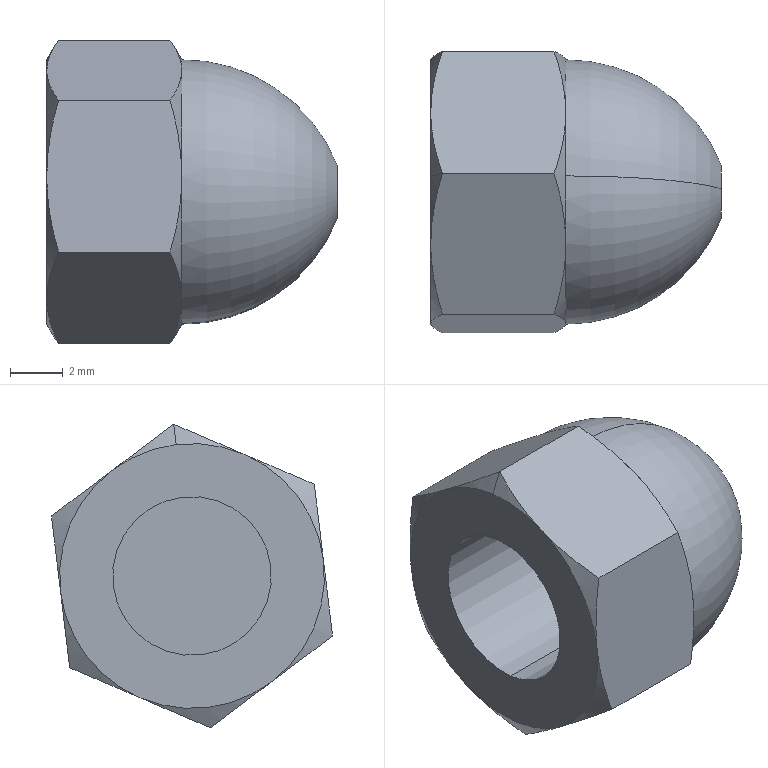Component | SolidWorks | DNR-71M20100BBEF2xx-A_990608MSS-1 | 1 solid | 26 faces | box 10.97 x 10.62 x 11.46 mm | volume 572 mm3 | cone 13 | plane 9 | torus 2 | cylinder 2 | commonest cylinder face diameters 6 x2
STEP:
#1=COLOUR_RGB('',0.7922,0.8196,0.9333);
#2=FILL_AREA_STYLE_COLOUR('',#1);
#3=FILL_AREA_STYLE('',(#2));
#4=SURFACE_STYLE_FILL_AREA(#3);
#5=SURFACE_SIDE_STYLE('',(#4));
#6=SURFACE_STYLE_USAGE(.BOTH.,#5);
#7=PRESENTATION_STYLE_ASSIGNMENT((#6));
#8=CARTESIAN_POINT('',(11.05,-7.185,8.11));
#9=VERTEX_POINT('',#8);
#10=CARTESIAN_POINT('',(11.05,-7.091,8.072));
#11=VERTEX_POINT('',#10);
#12=CARTESIAN_POINT('',(11.05,-7.067,8.267));
#13=DIRECTION('',(1.,-0.,-0.));
#14=DIRECTION('',(-0.,-0.9928,0.1196));
#15=AXIS2_PLACEMENT_3D('',#12,#13,#14);
#16=CIRCLE('',#15,0.1969);
#17=EDGE_CURVE('',#9,#11,#16,.T.);
#18=ORIENTED_EDGE('',*,*,#17,.T.);
#19=CARTESIAN_POINT('',(11.281,-7.072,8.227));
#20=VERTEX_POINT('',#19);
#21=CARTESIAN_POINT('',(11.05,-7.061,8.319));
#22=DIRECTION('',(-0.,-0.9928,0.1196));
#23=DIRECTION('',(0.,-0.1196,-0.9928));
#24=AXIS2_PLACEMENT_3D('',#21,#22,#23);
#25=CIRCLE('',#24,0.2487);
#26=EDGE_CURVE('',#11,#20,#25,.T.);
#27=ORIENTED_EDGE('',*,*,#26,.T.);
#28=CARTESIAN_POINT('',(11.281,-7.062,8.307));
#29=VERTEX_POINT('',#28);
#30=CARTESIAN_POINT('',(11.281,-7.067,8.267));
#31=DIRECTION('',(-1.,0.,0.));
#32=DIRECTION('',(0.,0.1196,0.9928));
#33=AXIS2_PLACEMENT_3D('',#30,#31,#32);
#34=CIRCLE('',#33,0.04003);
#35=EDGE_CURVE('',#20,#29,#34,.T.);
#36=ORIENTED_EDGE('',*,*,#35,.T.);
#37=CARTESIAN_POINT('',(11.05,-7.044,8.463));
#38=VERTEX_POINT('',#37);
#39=CARTESIAN_POINT('',(11.05,-7.073,8.216));
#40=DIRECTION('',(0.,0.9928,-0.1196));
#41=DIRECTION('',(0.,0.1196,0.9928));
#42=AXIS2_PLACEMENT_3D('',#39,#40,#41);
#43=CIRCLE('',#42,0.2487);
#44=EDGE_CURVE('',#38,#29,#43,.T.);
#45=ORIENTED_EDGE('',*,*,#44,.F.);
#46=CARTESIAN_POINT('',(11.05,-7.144,8.448));
#47=VERTEX_POINT('',#46);
#48=CARTESIAN_POINT('',(11.05,-7.067,8.267));
#49=DIRECTION('',(1.,0.,0.));
#50=DIRECTION('',(0.,-0.9928,0.1196));
#51=AXIS2_PLACEMENT_3D('',#48,#49,#50);
#52=CIRCLE('',#51,0.1969);
#53=EDGE_CURVE('',#38,#47,#52,.T.);
#54=ORIENTED_EDGE('',*,*,#53,.T.);
#55=CARTESIAN_POINT('',(11.05,-7.263,8.291));
#56=VERTEX_POINT('',#55);
#57=CARTESIAN_POINT('',(11.05,-7.067,8.267));
#58=DIRECTION('',(1.,0.,0.));
#59=DIRECTION('',(0.,-0.9928,0.1196));
#60=AXIS2_PLACEMENT_3D('',#57,#58,#59);
#61=CIRCLE('',#60,0.1969);
#62=EDGE_CURVE('',#47,#56,#61,.T.);
#63=ORIENTED_EDGE('',*,*,#62,.T.);
#64=CARTESIAN_POINT('',(11.05,-7.067,8.267));
#65=DIRECTION('',(1.,-0.,-0.));
#66=DIRECTION('',(-0.,-0.9928,0.1196));
#67=AXIS2_PLACEMENT_3D('',#64,#65,#66);
#68=CIRCLE('',#67,0.1969);
#69=EDGE_CURVE('',#56,#9,#68,.T.);
#70=ORIENTED_EDGE('',*,*,#69,.T.);
#71=EDGE_LOOP('',(#18,#27,#36,#45,#54,#63,#70));
#72=FACE_OUTER_BOUND('',#71,.T.);
#73=CARTESIAN_POINT('',(11.05,-7.067,8.267));
#74=DIRECTION('',(1.,-0.,-0.));
#75=DIRECTION('',(0.,0.1196,0.9928));
#76=AXIS2_PLACEMENT_3D('',#73,#74,#75);
#77=TOROIDAL_SURFACE('',#76,-0.05184,0.2487);
#78=ADVANCED_FACE('',(#72),#77,.T.);
#79=CARTESIAN_POINT('',(10.849,-6.949,8.425));
#80=VERTEX_POINT('',#79);
#81=CARTESIAN_POINT('',(10.849,-7.044,8.463));
#82=VERTEX_POINT('',#81);
#83=CARTESIAN_POINT('',(10.849,-7.067,8.267));
#84=DIRECTION('',(1.,-0.,-0.));
#85=DIRECTION('',(0.,0.1196,0.9928));
#86=AXIS2_PLACEMENT_3D('',#83,#84,#85);
#87=CIRCLE('',#86,0.1969);
#88=EDGE_CURVE('',#80,#82,#87,.T.);
#89=ORIENTED_EDGE('',*,*,#88,.T.);
#90=CARTESIAN_POINT('',(10.867,-7.04,8.493));
#91=VERTEX_POINT('',#90);
#92=CARTESIAN_POINT('',(10.867,-7.04,8.493));
#93=DIRECTION('',(0.5,0.1036,0.8598));
#94=VECTOR('',#93,39.37);
#95=LINE('',#92,#94);
#96=EDGE_CURVE('',#82,#91,#95,.T.);
#97=ORIENTED_EDGE('',*,*,#96,.T.);
#98=CARTESIAN_POINT('',(10.849,-6.949,8.425));
#99=CARTESIAN_POINT('',(10.849,-6.98,8.448));
#100=CARTESIAN_POINT('',(10.856,-7.01,8.47));
#101=CARTESIAN_POINT('',(10.867,-7.04,8.493));
#102=B_SPLINE_CURVE_WITH_KNOTS('',3,(#98,#99,#100,#101),.UNSPECIFIED.,.F.,.F.,(4,4),(0.,0.002921),.UNSPECIFIED.);
#103=EDGE_CURVE('',#80,#91,#102,.T.);
#104=ORIENTED_EDGE('',*,*,#103,.F.);
#105=EDGE_LOOP('',(#89,#97,#104));
#106=FACE_OUTER_BOUND('',#105,.T.);
#107=CARTESIAN_POINT('',(10.867,-7.067,8.267));
#108=DIRECTION('',(1.,-0.,-0.));
#109=DIRECTION('',(0.,0.1196,0.9928));
#110=AXIS2_PLACEMENT_3D('',#107,#108,#109);
#111=CONICAL_SURFACE('',#110,0.2275,1.047);
#112=ADVANCED_FACE('',(#106),#111,.T.);
#113=CARTESIAN_POINT('',(10.849,-7.081,8.15));
#114=VERTEX_POINT('',#113);
#115=CARTESIAN_POINT('',(10.849,-7.053,8.384));
#116=VERTEX_POINT('',#115);
#117=CARTESIAN_POINT('',(10.849,-7.067,8.267));
#118=DIRECTION('',(1.,-0.,-0.));
#119=DIRECTION('',(0.,0.1196,0.9928));
#120=AXIS2_PLACEMENT_3D('',#117,#118,#119);
#121=CIRCLE('',#120,0.1181);
#122=EDGE_CURVE('',#114,#116,#121,.T.);
#123=ORIENTED_EDGE('',*,*,#122,.F.);
#124=CARTESIAN_POINT('',(11.086,-7.081,8.15));
#125=VERTEX_POINT('',#124);
#126=CARTESIAN_POINT('',(10.849,-7.081,8.15));
#127=DIRECTION('',(1.,-0.,-0.));
#128=VECTOR('',#127,39.37);
#129=LINE('',#126,#128);
#130=EDGE_CURVE('',#114,#125,#129,.T.);
#131=ORIENTED_EDGE('',*,*,#130,.T.);
#132=CARTESIAN_POINT('',(11.086,-7.053,8.384));
#133=VERTEX_POINT('',#132);
#134=CARTESIAN_POINT('',(11.086,-7.067,8.267));
#135=DIRECTION('',(-1.,0.,0.));
#136=DIRECTION('',(0.,0.1196,0.9928));
#137=AXIS2_PLACEMENT_3D('',#134,#135,#136);
#138=CIRCLE('',#137,0.1181);
#139=EDGE_CURVE('',#133,#125,#138,.T.);
#140=ORIENTED_EDGE('',*,*,#139,.F.);
#141=CARTESIAN_POINT('',(10.849,-7.053,8.384));
#142=DIRECTION('',(1.,-0.,-0.));
#143=VECTOR('',#142,39.37);
#144=LINE('',#141,#143);
#145=EDGE_CURVE('',#116,#133,#144,.T.);
#146=ORIENTED_EDGE('',*,*,#145,.F.);
#147=EDGE_LOOP('',(#123,#131,#140,#146));
#148=FACE_OUTER_BOUND('',#147,.T.);
#149=CARTESIAN_POINT('',(10.849,-7.067,8.267));
#150=DIRECTION('',(1.,-0.,-0.));
#151=DIRECTION('',(0.,0.1196,0.9928));
#152=AXIS2_PLACEMENT_3D('',#149,#150,#151);
#153=CYLINDRICAL_SURFACE('',#152,0.1181);
#154=ADVANCED_FACE('',(#148),#153,.F.);
#155=ORIENTED_EDGE('',*,*,#26,.F.);
#156=CARTESIAN_POINT('',(11.05,-6.99,8.086));
#157=VERTEX_POINT('',#156);
#158=CARTESIAN_POINT('',(11.05,-7.067,8.267));
#159=DIRECTION('',(1.,-0.,-0.));
#160=DIRECTION('',(-0.,-0.9928,0.1196));
#161=AXIS2_PLACEMENT_3D('',#158,#159,#160);
#162=CIRCLE('',#161,0.1969);
#163=EDGE_CURVE('',#11,#157,#162,.T.);
#164=ORIENTED_EDGE('',*,*,#163,.T.);
#165=CARTESIAN_POINT('',(11.05,-6.872,8.244));
#166=VERTEX_POINT('',#165);
#167=CARTESIAN_POINT('',(11.05,-7.067,8.267));
#168=DIRECTION('',(1.,-0.,-0.));
#169=DIRECTION('',(-0.,-0.9928,0.1196));
#170=AXIS2_PLACEMENT_3D('',#167,#168,#169);
#171=CIRCLE('',#170,0.1969);
#172=EDGE_CURVE('',#157,#166,#171,.T.);
#173=ORIENTED_EDGE('',*,*,#172,.T.);
#174=CARTESIAN_POINT('',(11.05,-6.949,8.425));
#175=VERTEX_POINT('',#174);
#176=CARTESIAN_POINT('',(11.05,-7.067,8.267));
#177=DIRECTION('',(1.,0.,0.));
#178=DIRECTION('',(0.,-0.9928,0.1196));
#179=AXIS2_PLACEMENT_3D('',#176,#177,#178);
#180=CIRCLE('',#179,0.1969);
#181=EDGE_CURVE('',#166,#175,#180,.T.);
#182=ORIENTED_EDGE('',*,*,#181,.T.);
#183=CARTESIAN_POINT('',(11.05,-7.067,8.267));
#184=DIRECTION('',(1.,0.,0.));
#185=DIRECTION('',(0.,-0.9928,0.1196));
#186=AXIS2_PLACEMENT_3D('',#183,#184,#185);
#187=CIRCLE('',#186,0.1969);
#188=EDGE_CURVE('',#175,#38,#187,.T.);
#189=ORIENTED_EDGE('',*,*,#188,.T.);
#190=ORIENTED_EDGE('',*,*,#44,.T.);
#191=CARTESIAN_POINT('',(11.281,-7.067,8.267));
#192=DIRECTION('',(-1.,0.,0.));
#193=DIRECTION('',(0.,0.1196,0.9928));
#194=AXIS2_PLACEMENT_3D('',#191,#192,#193);
#195=CIRCLE('',#194,0.04003);
#196=EDGE_CURVE('',#29,#20,#195,.T.);
#197=ORIENTED_EDGE('',*,*,#196,.T.);
#198=EDGE_LOOP('',(#155,#164,#173,#182,#189,#190,#197));
#199=FACE_OUTER_BOUND('',#198,.T.);
#200=CARTESIAN_POINT('',(11.05,-7.067,8.267));
#201=DIRECTION('',(1.,-0.,-0.));
#202=DIRECTION('',(0.,0.1196,0.9928));
#203=AXIS2_PLACEMENT_3D('',#200,#201,#202);
#204=TOROIDAL_SURFACE('',#203,-0.05184,0.2487);
#205=ADVANCED_FACE('',(#199),#204,.T.);
#206=ORIENTED_EDGE('',*,*,#196,.F.);
#207=ORIENTED_EDGE('',*,*,#35,.F.);
#208=EDGE_LOOP('',(#206,#207));
#209=FACE_OUTER_BOUND('',#208,.T.);
#210=CARTESIAN_POINT('',(11.281,-7.067,8.267));
#211=DIRECTION('',(1.,-0.,-0.));
#212=DIRECTION('',(0.,0.1196,0.9928));
#213=AXIS2_PLACEMENT_3D('',#210,#211,#212);
#214=PLANE('',#213);
#215=ADVANCED_FACE('',(#209),#214,.T.);
#216=CARTESIAN_POINT('',(11.033,-6.885,8.131));
#217=VERTEX_POINT('',#216);
#218=CARTESIAN_POINT('',(11.033,-6.885,8.131));
#219=CARTESIAN_POINT('',(11.043,-6.881,8.168));
#220=CARTESIAN_POINT('',(11.05,-6.876,8.205));
#221=CARTESIAN_POINT('',(11.05,-6.872,8.244));
#222=B_SPLINE_CURVE_WITH_KNOTS('',3,(#218,#219,#220,#221),.UNSPECIFIED.,.F.,.F.,(4,4),(0.,0.002921),.UNSPECIFIED.);
#223=EDGE_CURVE('',#217,#166,#222,.T.);
#224=ORIENTED_EDGE('',*,*,#223,.T.);
#225=ORIENTED_EDGE('',*,*,#172,.F.);
#226=CARTESIAN_POINT('',(11.05,-6.99,8.086));
#227=CARTESIAN_POINT('',(11.05,-6.954,8.101));
#228=CARTESIAN_POINT('',(11.043,-6.919,8.116));
#229=CARTESIAN_POINT('',(11.033,-6.885,8.131));
#230=B_SPLINE_CURVE_WITH_KNOTS('',3,(#226,#227,#228,#229),.UNSPECIFIED.,.F.,.F.,(4,4),(0.,0.002921),.UNSPECIFIED.);
#231=EDGE_CURVE('',#157,#217,#230,.T.);
#232=ORIENTED_EDGE('',*,*,#231,.T.);
#233=EDGE_LOOP('',(#224,#225,#232));
#234=FACE_OUTER_BOUND('',#233,.T.);
#235=CARTESIAN_POINT('',(11.032,-7.067,8.267));
#236=DIRECTION('',(-1.,0.,0.));
#237=DIRECTION('',(0.,0.9928,-0.1196));
#238=AXIS2_PLACEMENT_3D('',#235,#236,#237);
#239=CONICAL_SURFACE('',#238,0.2275,1.047);
#240=ADVANCED_FACE('',(#234),#239,.T.);
#241=CARTESIAN_POINT('',(11.033,-7.094,8.041));
#242=VERTEX_POINT('',#241);
#243=CARTESIAN_POINT('',(11.033,-7.094,8.041));
#244=CARTESIAN_POINT('',(11.043,-7.06,8.056));
#245=CARTESIAN_POINT('',(11.05,-7.025,8.071));
#246=CARTESIAN_POINT('',(11.05,-6.99,8.086));
#247=B_SPLINE_CURVE_WITH_KNOTS('',3,(#243,#244,#245,#246),.UNSPECIFIED.,.F.,.F.,(4,4),(0.,0.002921),.UNSPECIFIED.);
#248=EDGE_CURVE('',#242,#157,#247,.T.);
#249=ORIENTED_EDGE('',*,*,#248,.T.);
#250=ORIENTED_EDGE('',*,*,#163,.F.);
#251=ORIENTED_EDGE('',*,*,#17,.F.);
#252=CARTESIAN_POINT('',(11.05,-7.185,8.11));
#253=CARTESIAN_POINT('',(11.05,-7.154,8.086));
#254=CARTESIAN_POINT('',(11.043,-7.124,8.064));
#255=CARTESIAN_POINT('',(11.033,-7.094,8.041));
#256=B_SPLINE_CURVE_WITH_KNOTS('',3,(#252,#253,#254,#255),.UNSPECIFIED.,.F.,.F.,(4,4),(0.,0.002921),.UNSPECIFIED.);
#257=EDGE_CURVE('',#9,#242,#256,.T.);
#258=ORIENTED_EDGE('',*,*,#257,.T.);
#259=EDGE_LOOP('',(#249,#250,#251,#258));
#260=FACE_OUTER_BOUND('',#259,.T.);
#261=CARTESIAN_POINT('',(11.032,-7.067,8.267));
#262=DIRECTION('',(-1.,0.,0.));
#263=DIRECTION('',(0.,0.9928,-0.1196));
#264=AXIS2_PLACEMENT_3D('',#261,#262,#263);
#265=CONICAL_SURFACE('',#264,0.2275,1.047);
#266=ADVANCED_FACE('',(#260),#265,.T.);
#267=CARTESIAN_POINT('',(11.033,-7.276,8.178));
#268=VERTEX_POINT('',#267);
#269=CARTESIAN_POINT('',(11.033,-7.276,8.178));
#270=CARTESIAN_POINT('',(11.043,-7.246,8.156));
#271=CARTESIAN_POINT('',(11.05,-7.216,8.133));
#272=CARTESIAN_POINT('',(11.05,-7.185,8.11));
#273=B_SPLINE_CURVE_WITH_KNOTS('',3,(#269,#270,#271,#272),.UNSPECIFIED.,.F.,.F.,(4,4),(0.,0.002921),.UNSPECIFIED.);
#274=EDGE_CURVE('',#268,#9,#273,.T.);
#275=ORIENTED_EDGE('',*,*,#274,.T.);
#276=ORIENTED_EDGE('',*,*,#69,.F.);
#277=CARTESIAN_POINT('',(11.05,-7.263,8.291));
#278=CARTESIAN_POINT('',(11.05,-7.267,8.252));
#279=CARTESIAN_POINT('',(11.043,-7.272,8.215));
#280=CARTESIAN_POINT('',(11.033,-7.276,8.178));
#281=B_SPLINE_CURVE_WITH_KNOTS('',3,(#277,#278,#279,#280),.UNSPECIFIED.,.F.,.F.,(4,4),(0.,0.002921),.UNSPECIFIED.);
#282=EDGE_CURVE('',#56,#268,#281,.T.);
#283=ORIENTED_EDGE('',*,*,#282,.T.);
#284=EDGE_LOOP('',(#275,#276,#283));
#285=FACE_OUTER_BOUND('',#284,.T.);
#286=CARTESIAN_POINT('',(11.032,-7.067,8.267));
#287=DIRECTION('',(-1.,0.,0.));
#288=DIRECTION('',(0.,0.9928,-0.1196));
#289=AXIS2_PLACEMENT_3D('',#286,#287,#288);
#290=CONICAL_SURFACE('',#289,0.2275,1.047);
#291=ADVANCED_FACE('',(#285),#290,.T.);
#292=CARTESIAN_POINT('',(11.033,-7.249,8.403));
#293=VERTEX_POINT('',#292);
#294=CARTESIAN_POINT('',(11.033,-7.249,8.403));
#295=CARTESIAN_POINT('',(11.043,-7.253,8.367));
#296=CARTESIAN_POINT('',(11.05,-7.258,8.329));
#297=CARTESIAN_POINT('',(11.05,-7.263,8.291));
#298=B_SPLINE_CURVE_WITH_KNOTS('',3,(#294,#295,#296,#297),.UNSPECIFIED.,.F.,.F.,(4,4),(0.,0.002921),.UNSPECIFIED.);
#299=EDGE_CURVE('',#293,#56,#298,.T.);
#300=ORIENTED_EDGE('',*,*,#299,.T.);
#301=ORIENTED_EDGE('',*,*,#62,.F.);
#302=CARTESIAN_POINT('',(11.05,-7.144,8.448));
#303=CARTESIAN_POINT('',(11.05,-7.18,8.433));
#304=CARTESIAN_POINT('',(11.043,-7.215,8.418));
#305=CARTESIAN_POINT('',(11.033,-7.249,8.403));
#306=B_SPLINE_CURVE_WITH_KNOTS('',3,(#302,#303,#304,#305),.UNSPECIFIED.,.F.,.F.,(4,4),(0.,0.002921),.UNSPECIFIED.);
#307=EDGE_CURVE('',#47,#293,#306,.T.);
#308=ORIENTED_EDGE('',*,*,#307,.T.);
#309=EDGE_LOOP('',(#300,#301,#308));
#310=FACE_OUTER_BOUND('',#309,.T.);
#311=CARTESIAN_POINT('',(11.032,-7.067,8.267));
#312=DIRECTION('',(-1.,0.,0.));
#313=DIRECTION('',(0.,0.9928,-0.1196));
#314=AXIS2_PLACEMENT_3D('',#311,#312,#313);
#315=CONICAL_SURFACE('',#314,0.2275,1.047);
#316=ADVANCED_FACE('',(#310),#315,.T.);
#317=CARTESIAN_POINT('',(11.033,-7.04,8.493));
#318=VERTEX_POINT('',#317);
#319=CARTESIAN_POINT('',(11.033,-7.04,8.493));
#320=CARTESIAN_POINT('',(11.043,-7.074,8.478));
#321=CARTESIAN_POINT('',(11.05,-7.109,8.463));
#322=CARTESIAN_POINT('',(11.05,-7.144,8.448));
#323=B_SPLINE_CURVE_WITH_KNOTS('',3,(#319,#320,#321,#322),.UNSPECIFIED.,.F.,.F.,(4,4),(0.,0.002921),.UNSPECIFIED.);
#324=EDGE_CURVE('',#318,#47,#323,.T.);
#325=ORIENTED_EDGE('',*,*,#324,.T.);
#326=ORIENTED_EDGE('',*,*,#53,.F.);
#327=ORIENTED_EDGE('',*,*,#188,.F.);
#328=CARTESIAN_POINT('',(11.05,-6.949,8.425));
#329=CARTESIAN_POINT('',(11.05,-6.98,8.448));
#330=CARTESIAN_POINT('',(11.043,-7.01,8.47));
#331=CARTESIAN_POINT('',(11.033,-7.04,8.493));
#332=B_SPLINE_CURVE_WITH_KNOTS('',3,(#328,#329,#330,#331),.UNSPECIFIED.,.F.,.F.,(4,4),(0.,0.002921),.UNSPECIFIED.);
#333=EDGE_CURVE('',#175,#318,#332,.T.);
#334=ORIENTED_EDGE('',*,*,#333,.T.);
#335=EDGE_LOOP('',(#325,#326,#327,#334));
#336=FACE_OUTER_BOUND('',#335,.T.);
#337=CARTESIAN_POINT('',(11.032,-7.067,8.267));
#338=DIRECTION('',(-1.,0.,0.));
#339=DIRECTION('',(0.,0.9928,-0.1196));
#340=AXIS2_PLACEMENT_3D('',#337,#338,#339);
#341=CONICAL_SURFACE('',#340,0.2275,1.047);
#342=ADVANCED_FACE('',(#336),#341,.T.);
#343=CARTESIAN_POINT('',(11.033,-6.858,8.356));
#344=VERTEX_POINT('',#343);
#345=CARTESIAN_POINT('',(11.033,-6.858,8.356));
#346=CARTESIAN_POINT('',(11.043,-6.888,8.379));
#347=CARTESIAN_POINT('',(11.05,-6.918,8.401));
#348=CARTESIAN_POINT('',(11.05,-6.949,8.425));
#349=B_SPLINE_CURVE_WITH_KNOTS('',3,(#345,#346,#347,#348),.UNSPECIFIED.,.F.,.F.,(4,4),(0.,0.002921),.UNSPECIFIED.);
#350=EDGE_CURVE('',#344,#175,#349,.T.);
#351=ORIENTED_EDGE('',*,*,#350,.T.);
#352=ORIENTED_EDGE('',*,*,#181,.F.);
#353=CARTESIAN_POINT('',(11.05,-6.872,8.244));
#354=CARTESIAN_POINT('',(11.05,-6.867,8.282));
#355=CARTESIAN_POINT('',(11.043,-6.862,8.32));
#356=CARTESIAN_POINT('',(11.033,-6.858,8.356));
#357=B_SPLINE_CURVE_WITH_KNOTS('',3,(#353,#354,#355,#356),.UNSPECIFIED.,.F.,.F.,(4,4),(0.,0.002921),.UNSPECIFIED.);
#358=EDGE_CURVE('',#166,#344,#357,.T.);
#359=ORIENTED_EDGE('',*,*,#358,.T.);
#360=EDGE_LOOP('',(#351,#352,#359));
#361=FACE_OUTER_BOUND('',#360,.T.);
#362=CARTESIAN_POINT('',(11.032,-7.067,8.267));
#363=DIRECTION('',(-1.,0.,0.));
#364=DIRECTION('',(0.,0.9928,-0.1196));
#365=AXIS2_PLACEMENT_3D('',#362,#363,#364);
#366=CONICAL_SURFACE('',#365,0.2275,1.047);
#367=ADVANCED_FACE('',(#361),#366,.T.);
#368=CARTESIAN_POINT('',(10.867,-6.858,8.356));
#369=VERTEX_POINT('',#368);
#370=CARTESIAN_POINT('',(11.05,-6.858,8.356));
#371=DIRECTION('',(1.,-0.,-0.));
#372=VECTOR('',#371,39.37);
#373=LINE('',#370,#372);
#374=EDGE_CURVE('',#369,#344,#373,.T.);
#375=ORIENTED_EDGE('',*,*,#374,.T.);
#376=ORIENTED_EDGE('',*,*,#358,.F.);
#377=ORIENTED_EDGE('',*,*,#223,.F.);
#378=CARTESIAN_POINT('',(10.867,-6.885,8.131));
#379=VERTEX_POINT('',#378);
#380=CARTESIAN_POINT('',(11.05,-6.885,8.131));
#381=DIRECTION('',(-1.,0.,0.));
#382=VECTOR('',#381,39.37);
#383=LINE('',#380,#382);
#384=EDGE_CURVE('',#217,#379,#383,.T.);
#385=ORIENTED_EDGE('',*,*,#384,.T.);
#386=CARTESIAN_POINT('',(10.849,-6.872,8.244));
#387=VERTEX_POINT('',#386);
#388=CARTESIAN_POINT('',(10.867,-6.885,8.131));
#389=CARTESIAN_POINT('',(10.856,-6.881,8.168));
#390=CARTESIAN_POINT('',(10.849,-6.876,8.205));
#391=CARTESIAN_POINT('',(10.849,-6.872,8.244));
#392=B_SPLINE_CURVE_WITH_KNOTS('',3,(#388,#389,#390,#391),.UNSPECIFIED.,.F.,.F.,(4,4),(0.,0.002921),.UNSPECIFIED.);
#393=EDGE_CURVE('',#379,#387,#392,.T.);
#394=ORIENTED_EDGE('',*,*,#393,.T.);
#395=CARTESIAN_POINT('',(10.849,-6.872,8.244));
#396=CARTESIAN_POINT('',(10.849,-6.867,8.282));
#397=CARTESIAN_POINT('',(10.856,-6.862,8.32));
#398=CARTESIAN_POINT('',(10.867,-6.858,8.356));
#399=B_SPLINE_CURVE_WITH_KNOTS('',3,(#395,#396,#397,#398),.UNSPECIFIED.,.F.,.F.,(4,4),(0.,0.002921),.UNSPECIFIED.);
#400=EDGE_CURVE('',#387,#369,#399,.T.);
#401=ORIENTED_EDGE('',*,*,#400,.T.);
#402=EDGE_LOOP('',(#375,#376,#377,#385,#394,#401));
#403=FACE_OUTER_BOUND('',#402,.T.);
#404=CARTESIAN_POINT('',(11.05,-6.858,8.356));
#405=DIRECTION('',(0.,0.9928,-0.1196));
#406=DIRECTION('',(1.,-0.,-0.));
#407=AXIS2_PLACEMENT_3D('',#404,#405,#406);
#408=PLANE('',#407);
#409=ADVANCED_FACE('',(#403),#408,.T.);
#410=ORIENTED_EDGE('',*,*,#384,.F.);
#411=ORIENTED_EDGE('',*,*,#231,.F.);
#412=ORIENTED_EDGE('',*,*,#248,.F.);
#413=CARTESIAN_POINT('',(10.867,-7.094,8.041));
#414=VERTEX_POINT('',#413);
#415=CARTESIAN_POINT('',(11.05,-7.094,8.041));
#416=DIRECTION('',(-1.,0.,0.));
#417=VECTOR('',#416,39.37);
#418=LINE('',#415,#417);
#419=EDGE_CURVE('',#242,#414,#418,.T.);
#420=ORIENTED_EDGE('',*,*,#419,.T.);
#421=CARTESIAN_POINT('',(10.849,-6.99,8.086));
#422=VERTEX_POINT('',#421);
#423=CARTESIAN_POINT('',(10.867,-7.094,8.041));
#424=CARTESIAN_POINT('',(10.856,-7.06,8.056));
#425=CARTESIAN_POINT('',(10.849,-7.025,8.071));
#426=CARTESIAN_POINT('',(10.849,-6.99,8.086));
#427=B_SPLINE_CURVE_WITH_KNOTS('',3,(#423,#424,#425,#426),.UNSPECIFIED.,.F.,.F.,(4,4),(0.,0.002921),.UNSPECIFIED.);
#428=EDGE_CURVE('',#414,#422,#427,.T.);
#429=ORIENTED_EDGE('',*,*,#428,.T.);
#430=CARTESIAN_POINT('',(10.849,-6.99,8.086));
#431=CARTESIAN_POINT('',(10.849,-6.954,8.101));
#432=CARTESIAN_POINT('',(10.856,-6.919,8.116));
#433=CARTESIAN_POINT('',(10.867,-6.885,8.131));
#434=B_SPLINE_CURVE_WITH_KNOTS('',3,(#430,#431,#432,#433),.UNSPECIFIED.,.F.,.F.,(4,4),(0.,0.002921),.UNSPECIFIED.);
#435=EDGE_CURVE('',#422,#379,#434,.T.);
#436=ORIENTED_EDGE('',*,*,#435,.T.);
#437=EDGE_LOOP('',(#410,#411,#412,#420,#429,#436));
#438=FACE_OUTER_BOUND('',#437,.T.);
#439=CARTESIAN_POINT('',(11.05,-6.885,8.131));
#440=DIRECTION('',(-0.,0.3928,-0.9196));
#441=DIRECTION('',(-0.,-0.9196,-0.3928));
#442=AXIS2_PLACEMENT_3D('',#439,#440,#441);
#443=PLANE('',#442);
#444=ADVANCED_FACE('',(#438),#443,.T.);
#445=ORIENTED_EDGE('',*,*,#419,.F.);
#446=ORIENTED_EDGE('',*,*,#257,.F.);
#447=ORIENTED_EDGE('',*,*,#274,.F.);
#448=CARTESIAN_POINT('',(10.867,-7.276,8.178));
#449=VERTEX_POINT('',#448);
#450=CARTESIAN_POINT('',(11.05,-7.276,8.178));
#451=DIRECTION('',(-1.,0.,0.));
#452=VECTOR('',#451,39.37);
#453=LINE('',#450,#452);
#454=EDGE_CURVE('',#268,#449,#453,.T.);
#455=ORIENTED_EDGE('',*,*,#454,.T.);
#456=CARTESIAN_POINT('',(10.849,-7.185,8.11));
#457=VERTEX_POINT('',#456);
#458=CARTESIAN_POINT('',(10.867,-7.276,8.178));
#459=CARTESIAN_POINT('',(10.856,-7.246,8.156));
#460=CARTESIAN_POINT('',(10.849,-7.216,8.133));
#461=CARTESIAN_POINT('',(10.849,-7.185,8.11));
#462=B_SPLINE_CURVE_WITH_KNOTS('',3,(#458,#459,#460,#461),.UNSPECIFIED.,.F.,.F.,(4,4),(0.,0.002921),.UNSPECIFIED.);
#463=EDGE_CURVE('',#449,#457,#462,.T.);
#464=ORIENTED_EDGE('',*,*,#463,.T.);
#465=CARTESIAN_POINT('',(10.849,-7.185,8.11));
#466=CARTESIAN_POINT('',(10.849,-7.154,8.086));
#467=CARTESIAN_POINT('',(10.856,-7.124,8.064));
#468=CARTESIAN_POINT('',(10.867,-7.094,8.041));
#469=B_SPLINE_CURVE_WITH_KNOTS('',3,(#465,#466,#467,#468),.UNSPECIFIED.,.F.,.F.,(4,4),(0.,0.002921),.UNSPECIFIED.);
#470=EDGE_CURVE('',#457,#414,#469,.T.);
#471=ORIENTED_EDGE('',*,*,#470,.T.);
#472=EDGE_LOOP('',(#445,#446,#447,#455,#464,#471));
#473=FACE_OUTER_BOUND('',#472,.T.);
#474=CARTESIAN_POINT('',(11.05,-7.094,8.041));
#475=DIRECTION('',(-0.,-0.6,-0.8));
#476=DIRECTION('',(-0.,-0.8,0.6));
#477=AXIS2_PLACEMENT_3D('',#474,#475,#476);
#478=PLANE('',#477);
#479=ADVANCED_FACE('',(#473),#478,.T.);
#480=ORIENTED_EDGE('',*,*,#454,.F.);
#481=ORIENTED_EDGE('',*,*,#282,.F.);
#482=ORIENTED_EDGE('',*,*,#299,.F.);
#483=CARTESIAN_POINT('',(10.867,-7.249,8.403));
#484=VERTEX_POINT('',#483);
#485=CARTESIAN_POINT('',(11.05,-7.249,8.403));
#486=DIRECTION('',(-1.,0.,0.));
#487=VECTOR('',#486,39.37);
#488=LINE('',#485,#487);
#489=EDGE_CURVE('',#293,#484,#488,.T.);
#490=ORIENTED_EDGE('',*,*,#489,.T.);
#491=CARTESIAN_POINT('',(10.849,-7.263,8.291));
#492=VERTEX_POINT('',#491);
#493=CARTESIAN_POINT('',(10.867,-7.249,8.403));
#494=CARTESIAN_POINT('',(10.856,-7.253,8.367));
#495=CARTESIAN_POINT('',(10.849,-7.258,8.329));
#496=CARTESIAN_POINT('',(10.849,-7.263,8.291));
#497=B_SPLINE_CURVE_WITH_KNOTS('',3,(#493,#494,#495,#496),.UNSPECIFIED.,.F.,.F.,(4,4),(0.,0.002921),.UNSPECIFIED.);
#498=EDGE_CURVE('',#484,#492,#497,.T.);
#499=ORIENTED_EDGE('',*,*,#498,.T.);
#500=CARTESIAN_POINT('',(10.849,-7.263,8.291));
#501=CARTESIAN_POINT('',(10.849,-7.267,8.252));
#502=CARTESIAN_POINT('',(10.856,-7.272,8.215));
#503=CARTESIAN_POINT('',(10.867,-7.276,8.178));
#504=B_SPLINE_CURVE_WITH_KNOTS('',3,(#500,#501,#502,#503),.UNSPECIFIED.,.F.,.F.,(4,4),(0.,0.002921),.UNSPECIFIED.);
#505=EDGE_CURVE('',#492,#449,#504,.T.);
#506=ORIENTED_EDGE('',*,*,#505,.T.);
#507=EDGE_LOOP('',(#480,#481,#482,#490,#499,#506));
#508=FACE_OUTER_BOUND('',#507,.T.);
#509=CARTESIAN_POINT('',(11.05,-7.276,8.178));
#510=DIRECTION('',(-0.,-0.9928,0.1196));
#511=DIRECTION('',(-1.,0.,0.));
#512=AXIS2_PLACEMENT_3D('',#509,#510,#511);
#513=PLANE('',#512);
#514=ADVANCED_FACE('',(#508),#513,.T.);
#515=ORIENTED_EDGE('',*,*,#489,.F.);
#516=ORIENTED_EDGE('',*,*,#307,.F.);
#517=ORIENTED_EDGE('',*,*,#324,.F.);
#518=CARTESIAN_POINT('',(11.05,-7.04,8.493));
#519=DIRECTION('',(-1.,0.,0.));
#520=VECTOR('',#519,39.37);
#521=LINE('',#518,#520);
#522=EDGE_CURVE('',#318,#91,#521,.T.);
#523=ORIENTED_EDGE('',*,*,#522,.T.);
#524=CARTESIAN_POINT('',(10.849,-7.144,8.448));
#525=VERTEX_POINT('',#524);
#526=CARTESIAN_POINT('',(10.867,-7.04,8.493));
#527=CARTESIAN_POINT('',(10.856,-7.074,8.478));
#528=CARTESIAN_POINT('',(10.849,-7.109,8.463));
#529=CARTESIAN_POINT('',(10.849,-7.144,8.448));
#530=B_SPLINE_CURVE_WITH_KNOTS('',3,(#526,#527,#528,#529),.UNSPECIFIED.,.F.,.F.,(4,4),(0.,0.002921),.UNSPECIFIED.);
#531=EDGE_CURVE('',#91,#525,#530,.T.);
#532=ORIENTED_EDGE('',*,*,#531,.T.);
#533=CARTESIAN_POINT('',(10.849,-7.144,8.448));
#534=CARTESIAN_POINT('',(10.849,-7.18,8.433));
#535=CARTESIAN_POINT('',(10.856,-7.215,8.418));
#536=CARTESIAN_POINT('',(10.867,-7.249,8.403));
#537=B_SPLINE_CURVE_WITH_KNOTS('',3,(#533,#534,#535,#536),.UNSPECIFIED.,.F.,.F.,(4,4),(0.,0.002921),.UNSPECIFIED.);
#538=EDGE_CURVE('',#525,#484,#537,.T.);
#539=ORIENTED_EDGE('',*,*,#538,.T.);
#540=EDGE_LOOP('',(#515,#516,#517,#523,#532,#539));
#541=FACE_OUTER_BOUND('',#540,.T.);
#542=CARTESIAN_POINT('',(11.05,-7.249,8.403));
#543=DIRECTION('',(0.,-0.3928,0.9196));
#544=DIRECTION('',(0.,0.9196,0.3928));
#545=AXIS2_PLACEMENT_3D('',#542,#543,#544);
#546=PLANE('',#545);
#547=ADVANCED_FACE('',(#541),#546,.T.);
#548=ORIENTED_EDGE('',*,*,#522,.F.);
#549=ORIENTED_EDGE('',*,*,#333,.F.);
#550=ORIENTED_EDGE('',*,*,#350,.F.);
#551=ORIENTED_EDGE('',*,*,#374,.F.);
#552=CARTESIAN_POINT('',(10.867,-6.858,8.356));
#553=CARTESIAN_POINT('',(10.856,-6.888,8.379));
#554=CARTESIAN_POINT('',(10.849,-6.918,8.401));
#555=CARTESIAN_POINT('',(10.849,-6.949,8.425));
#556=B_SPLINE_CURVE_WITH_KNOTS('',3,(#552,#553,#554,#555),.UNSPECIFIED.,.F.,.F.,(4,4),(0.,0.002921),.UNSPECIFIED.);
#557=EDGE_CURVE('',#369,#80,#556,.T.);
#558=ORIENTED_EDGE('',*,*,#557,.T.);
#559=ORIENTED_EDGE('',*,*,#103,.T.);
#560=EDGE_LOOP('',(#548,#549,#550,#551,#558,#559));
#561=FACE_OUTER_BOUND('',#560,.T.);
#562=CARTESIAN_POINT('',(11.05,-7.04,8.493));
#563=DIRECTION('',(0.,0.6,0.8));
#564=DIRECTION('',(0.,0.8,-0.6));
#565=AXIS2_PLACEMENT_3D('',#562,#563,#564);
#566=PLANE('',#565);
#567=ADVANCED_FACE('',(#561),#566,.T.);
#568=ORIENTED_EDGE('',*,*,#400,.F.);
#569=CARTESIAN_POINT('',(10.849,-7.067,8.267));
#570=DIRECTION('',(1.,-0.,-0.));
#571=DIRECTION('',(0.,0.1196,0.9928));
#572=AXIS2_PLACEMENT_3D('',#569,#570,#571);
#573=CIRCLE('',#572,0.1969);
#574=EDGE_CURVE('',#387,#80,#573,.T.);
#575=ORIENTED_EDGE('',*,*,#574,.T.);
#576=ORIENTED_EDGE('',*,*,#557,.F.);
#577=EDGE_LOOP('',(#568,#575,#576));
#578=FACE_OUTER_BOUND('',#577,.T.);
#579=CARTESIAN_POINT('',(10.867,-7.067,8.267));
#580=DIRECTION('',(1.,-0.,-0.));
#581=DIRECTION('',(0.,0.1196,0.9928));
#582=AXIS2_PLACEMENT_3D('',#579,#580,#581);
#583=CONICAL_SURFACE('',#582,0.2275,1.047);
#584=ADVANCED_FACE('',(#578),#583,.T.);
#585=ORIENTED_EDGE('',*,*,#435,.F.);
#586=CARTESIAN_POINT('',(10.849,-7.067,8.267));
#587=DIRECTION('',(1.,-0.,-0.));
#588=DIRECTION('',(0.,0.1196,0.9928));
#589=AXIS2_PLACEMENT_3D('',#586,#587,#588);
#590=CIRCLE('',#589,0.1969);
#591=EDGE_CURVE('',#422,#387,#590,.T.);
#592=ORIENTED_EDGE('',*,*,#591,.T.);
#593=ORIENTED_EDGE('',*,*,#393,.F.);
#594=EDGE_LOOP('',(#585,#592,#593));
#595=FACE_OUTER_BOUND('',#594,.T.);
#596=CARTESIAN_POINT('',(10.867,-7.067,8.267));
#597=DIRECTION('',(1.,-0.,-0.));
#598=DIRECTION('',(0.,0.1196,0.9928));
#599=AXIS2_PLACEMENT_3D('',#596,#597,#598);
#600=CONICAL_SURFACE('',#599,0.2275,1.047);
#601=ADVANCED_FACE('',(#595),#600,.T.);
#602=ORIENTED_EDGE('',*,*,#470,.F.);
#603=CARTESIAN_POINT('',(10.849,-7.067,8.267));
#604=DIRECTION('',(1.,-0.,-0.));
#605=DIRECTION('',(0.,0.1196,0.9928));
#606=AXIS2_PLACEMENT_3D('',#603,#604,#605);
#607=CIRCLE('',#606,0.1969);
#608=EDGE_CURVE('',#457,#422,#607,.T.);
#609=ORIENTED_EDGE('',*,*,#608,.T.);
#610=ORIENTED_EDGE('',*,*,#428,.F.);
#611=EDGE_LOOP('',(#602,#609,#610));
#612=FACE_OUTER_BOUND('',#611,.T.);
#613=CARTESIAN_POINT('',(10.867,-7.067,8.267));
#614=DIRECTION('',(1.,-0.,-0.));
#615=DIRECTION('',(0.,0.1196,0.9928));
#616=AXIS2_PLACEMENT_3D('',#613,#614,#615);
#617=CONICAL_SURFACE('',#616,0.2275,1.047);
#618=ADVANCED_FACE('',(#612),#617,.T.);
#619=ORIENTED_EDGE('',*,*,#505,.F.);
#620=CARTESIAN_POINT('',(10.849,-7.067,8.267));
#621=DIRECTION('',(1.,-0.,-0.));
#622=DIRECTION('',(0.,0.1196,0.9928));
#623=AXIS2_PLACEMENT_3D('',#620,#621,#622);
#624=CIRCLE('',#623,0.1969);
#625=EDGE_CURVE('',#492,#457,#624,.T.);
#626=ORIENTED_EDGE('',*,*,#625,.T.);
#627=ORIENTED_EDGE('',*,*,#463,.F.);
#628=EDGE_LOOP('',(#619,#626,#627));
#629=FACE_OUTER_BOUND('',#628,.T.);
#630=CARTESIAN_POINT('',(10.867,-7.067,8.267));
#631=DIRECTION('',(1.,-0.,-0.));
#632=DIRECTION('',(0.,0.1196,0.9928));
#633=AXIS2_PLACEMENT_3D('',#630,#631,#632);
#634=CONICAL_SURFACE('',#633,0.2275,1.047);
#635=ADVANCED_FACE('',(#629),#634,.T.);
#636=ORIENTED_EDGE('',*,*,#538,.F.);
#637=CARTESIAN_POINT('',(10.849,-7.067,8.267));
#638=DIRECTION('',(1.,-0.,-0.));
#639=DIRECTION('',(0.,0.1196,0.9928));
#640=AXIS2_PLACEMENT_3D('',#637,#638,#639);
#641=CIRCLE('',#640,0.1969);
#642=EDGE_CURVE('',#525,#492,#641,.T.);
#643=ORIENTED_EDGE('',*,*,#642,.T.);
#644=ORIENTED_EDGE('',*,*,#498,.F.);
#645=EDGE_LOOP('',(#636,#643,#644));
#646=FACE_OUTER_BOUND('',#645,.T.);
#647=CARTESIAN_POINT('',(10.867,-7.067,8.267));
#648=DIRECTION('',(1.,-0.,-0.));
#649=DIRECTION('',(0.,0.1196,0.9928));
#650=AXIS2_PLACEMENT_3D('',#647,#648,#649);
#651=CONICAL_SURFACE('',#650,0.2275,1.047);
#652=ADVANCED_FACE('',(#646),#651,.T.);
#653=ORIENTED_EDGE('',*,*,#96,.F.);
#654=CARTESIAN_POINT('',(10.849,-7.067,8.267));
#655=DIRECTION('',(1.,-0.,-0.));
#656=DIRECTION('',(0.,0.1196,0.9928));
#657=AXIS2_PLACEMENT_3D('',#654,#655,#656);
#658=CIRCLE('',#657,0.1969);
#659=EDGE_CURVE('',#82,#525,#658,.T.);
#660=ORIENTED_EDGE('',*,*,#659,.T.);
#661=ORIENTED_EDGE('',*,*,#531,.F.);
#662=EDGE_LOOP('',(#653,#660,#661));
#663=FACE_OUTER_BOUND('',#662,.T.);
#664=CARTESIAN_POINT('',(10.867,-7.067,8.267));
#665=DIRECTION('',(1.,-0.,-0.));
#666=DIRECTION('',(0.,0.1196,0.9928));
#667=AXIS2_PLACEMENT_3D('',#664,#665,#666);
#668=CONICAL_SURFACE('',#667,0.2275,1.047);
#669=ADVANCED_FACE('',(#663),#668,.T.);
#670=CARTESIAN_POINT('',(10.849,-7.067,8.267));
#671=DIRECTION('',(1.,-0.,-0.));
#672=DIRECTION('',(0.,0.1196,0.9928));
#673=AXIS2_PLACEMENT_3D('',#670,#671,#672);
#674=CIRCLE('',#673,0.1181);
#675=EDGE_CURVE('',#116,#114,#674,.T.);
#676=ORIENTED_EDGE('',*,*,#675,.T.);
#677=ORIENTED_EDGE('',*,*,#122,.T.);
#678=EDGE_LOOP('',(#676,#677));
#679=FACE_BOUND('',#678,.T.);
#680=ORIENTED_EDGE('',*,*,#591,.F.);
#681=ORIENTED_EDGE('',*,*,#608,.F.);
#682=ORIENTED_EDGE('',*,*,#625,.F.);
#683=ORIENTED_EDGE('',*,*,#642,.F.);
#684=ORIENTED_EDGE('',*,*,#659,.F.);
#685=ORIENTED_EDGE('',*,*,#88,.F.);
#686=ORIENTED_EDGE('',*,*,#574,.F.);
#687=EDGE_LOOP('',(#680,#681,#682,#683,#684,#685,#686));
#688=FACE_OUTER_BOUND('',#687,.T.);
#689=CARTESIAN_POINT('',(10.849,-7.067,8.267));
#690=DIRECTION('',(-1.,0.,0.));
#691=DIRECTION('',(-0.,-0.1196,-0.9928));
#692=AXIS2_PLACEMENT_3D('',#689,#690,#691);
#693=PLANE('',#692);
#694=ADVANCED_FACE('',(#679,#688),#693,.T.);
#695=ORIENTED_EDGE('',*,*,#130,.F.);
#696=ORIENTED_EDGE('',*,*,#675,.F.);
#697=ORIENTED_EDGE('',*,*,#145,.T.);
#698=CARTESIAN_POINT('',(11.086,-7.067,8.267));
#699=DIRECTION('',(-1.,0.,0.));
#700=DIRECTION('',(0.,0.1196,0.9928));
#701=AXIS2_PLACEMENT_3D('',#698,#699,#700);
#702=CIRCLE('',#701,0.1181);
#703=EDGE_CURVE('',#125,#133,#702,.T.);
#704=ORIENTED_EDGE('',*,*,#703,.F.);
#705=EDGE_LOOP('',(#695,#696,#697,#704));
#706=FACE_OUTER_BOUND('',#705,.T.);
#707=CARTESIAN_POINT('',(10.849,-7.067,8.267));
#708=DIRECTION('',(1.,-0.,-0.));
#709=DIRECTION('',(0.,0.1196,0.9928));
#710=AXIS2_PLACEMENT_3D('',#707,#708,#709);
#711=CYLINDRICAL_SURFACE('',#710,0.1181);
#712=ADVANCED_FACE('',(#706),#711,.F.);
#713=ORIENTED_EDGE('',*,*,#139,.T.);
#714=ORIENTED_EDGE('',*,*,#703,.T.);
#715=EDGE_LOOP('',(#713,#714));
#716=FACE_OUTER_BOUND('',#715,.T.);
#717=CARTESIAN_POINT('',(11.086,-7.067,8.267));
#718=DIRECTION('',(1.,-0.,-0.));
#719=DIRECTION('',(0.,0.1196,0.9928));
#720=AXIS2_PLACEMENT_3D('',#717,#718,#719);
#721=PLANE('',#720);
#722=ADVANCED_FACE('',(#716),#721,.F.);
#723=CLOSED_SHELL('',(#78,#112,#154,#205,#215,#240,#266,#291,#316,#342,#367,#409,#444,#479,#514,#547,#567,#584,#601,#618,#635,#652,#669,#694,#712,#722));
#724=MANIFOLD_SOLID_BREP('',#723);
#725=STYLED_ITEM('',(#7),#724);
#726=(LENGTH_UNIT()NAMED_UNIT(*)SI_UNIT($,.METRE.));
#727=LENGTH_MEASURE_WITH_UNIT(LENGTH_MEASURE(0.0254),#726);
#728=DIMENSIONAL_EXPONENTS(1.,0.,0.,0.,0.,0.,0.);
#729=(CONVERSION_BASED_UNIT('',#727)LENGTH_UNIT()NAMED_UNIT(#728));
#730=UNCERTAINTY_MEASURE_WITH_UNIT(LENGTH_MEASURE(0.00001),#729,'','');
#731=(NAMED_UNIT(*)PLANE_ANGLE_UNIT()SI_UNIT($,.RADIAN.));
#732=(NAMED_UNIT(*)SI_UNIT($,.STERADIAN.)SOLID_ANGLE_UNIT());
#733=(GEOMETRIC_REPRESENTATION_CONTEXT(3)GLOBAL_UNCERTAINTY_ASSIGNED_CONTEXT((#730))GLOBAL_UNIT_ASSIGNED_CONTEXT((#729,#731,#732))REPRESENTATION_CONTEXT('',''));
#734=MECHANICAL_DESIGN_GEOMETRIC_PRESENTATION_REPRESENTATION('',(#725),#733);
#735=PRESENTATION_LAYER_ASSIGNMENT('','',(#725));
#736=CARTESIAN_POINT('',(0.,0.,0.));
#737=DIRECTION('',(0.,0.,1.));
#738=DIRECTION('',(1.,0.,0.));
#739=AXIS2_PLACEMENT_3D('',#736,#737,#738);
#740=(LENGTH_UNIT()NAMED_UNIT(*)SI_UNIT($,.METRE.));
#741=LENGTH_MEASURE_WITH_UNIT(LENGTH_MEASURE(0.0254),#740);
#742=DIMENSIONAL_EXPONENTS(1.,0.,0.,0.,0.,0.,0.);
#743=(CONVERSION_BASED_UNIT('',#741)LENGTH_UNIT()NAMED_UNIT(#742));
#744=UNCERTAINTY_MEASURE_WITH_UNIT(LENGTH_MEASURE(0.00001),#743,'','');
#745=(NAMED_UNIT(*)PLANE_ANGLE_UNIT()SI_UNIT($,.RADIAN.));
#746=(NAMED_UNIT(*)SI_UNIT($,.STERADIAN.)SOLID_ANGLE_UNIT());
#747=(GEOMETRIC_REPRESENTATION_CONTEXT(3)GLOBAL_UNCERTAINTY_ASSIGNED_CONTEXT((#744))GLOBAL_UNIT_ASSIGNED_CONTEXT((#743,#745,#746))REPRESENTATION_CONTEXT('',''));
#748=ADVANCED_BREP_SHAPE_REPRESENTATION('',(#724,#739),#747);